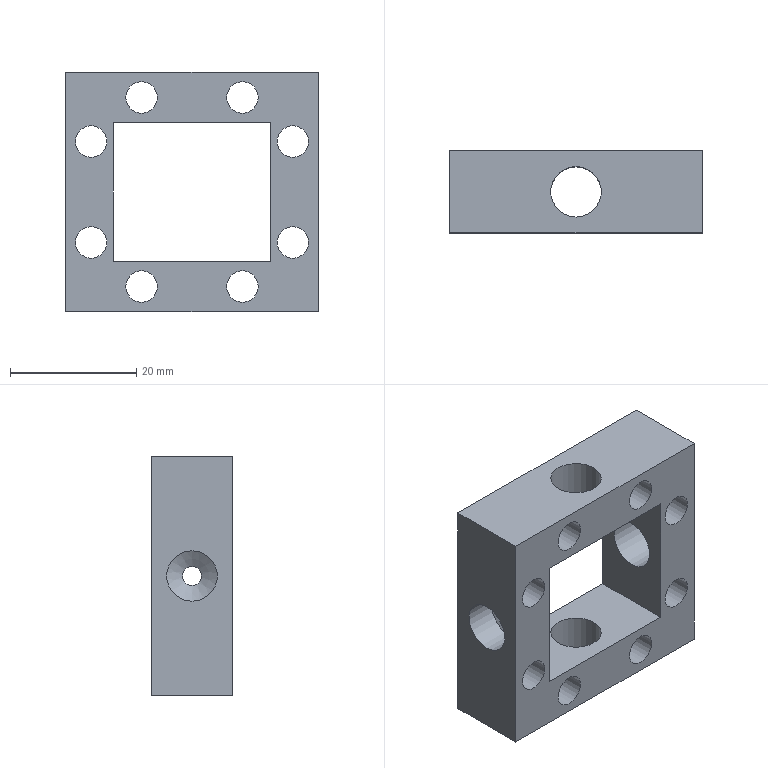Component | NX | EXTERNAL_PISTON_CYLINDER_BODY | 1 solid | 24 faces | volume 9090 mm3 | cylinder 13 | plane 10 | cone 1 | commonest cylinder face diameters 5 x8 8 x4 3 x1